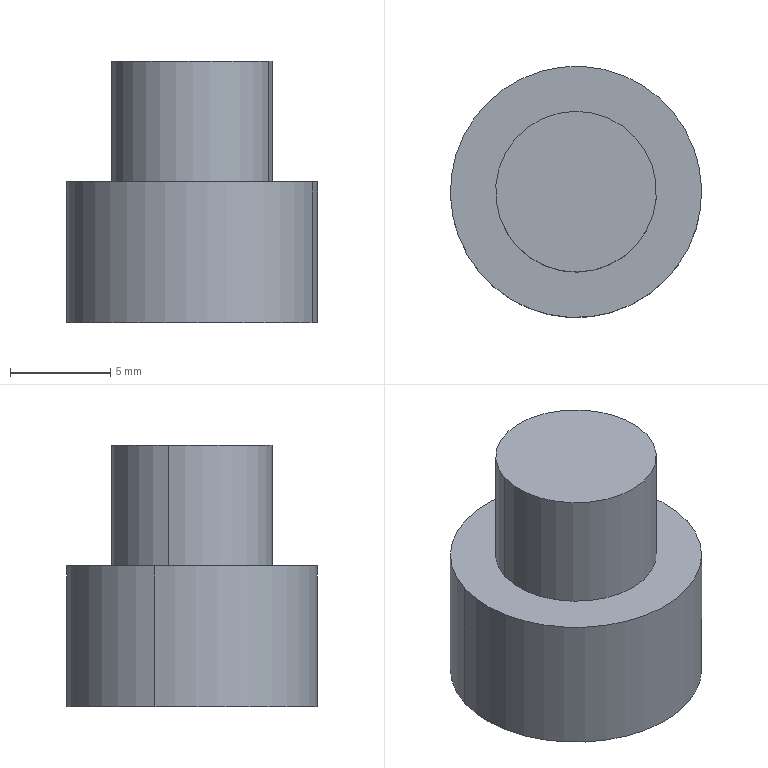Component | SolidWorks | PER_N-1 | 1 solid | 7 faces | box 12.5 x 12.5 x 13 mm | volume 1161 mm3 | cylinder 4 | plane 3 | commonest cylinder face diameters 8 x2 12.5 x2
build123d program:
from build123d import *

# Parameters (mm, degrees)
IZIM1_R                     = 6.25
Y_KSEKLIK_EKSTR_ZYON1_DEPTH = 7
IZIM2_R                     = 4
Y_KSEKLIK_EKSTR_ZYON2_DEPTH = 6


with BuildPart() as part:
    # izim1 → Y_kseklik-Ekstr_zyon1 (new body)
    with BuildSketch(Plane.XY):
        Circle(IZIM1_R)
    extrude(amount=Y_KSEKLIK_EKSTR_ZYON1_DEPTH)

    # izim2 → Y_kseklik-Ekstr_zyon2 (add)
    with BuildSketch(Plane.XY.offset(7)):
        Circle(IZIM2_R)
    extrude(amount=Y_KSEKLIK_EKSTR_ZYON2_DEPTH)


solid = part.part

# Placed as in the assembly
solid = solid.moved(Location((-146.473, 169.805, 173.974), (0, 0, 0)))
STEP:
#1=COLOUR_RGB('',0.7922,0.8196,0.9333);
#2=FILL_AREA_STYLE_COLOUR('',#1);
#3=FILL_AREA_STYLE('',(#2));
#4=SURFACE_STYLE_FILL_AREA(#3);
#5=SURFACE_SIDE_STYLE('',(#4));
#6=SURFACE_STYLE_USAGE(.BOTH.,#5);
#7=PRESENTATION_STYLE_ASSIGNMENT((#6));
#8=CARTESIAN_POINT('',(-5.917,6.732,7.361));
#9=VERTEX_POINT('',#8);
#10=CARTESIAN_POINT('',(-5.616,6.639,7.361));
#11=VERTEX_POINT('',#10);
#12=CARTESIAN_POINT('',(-5.767,6.685,7.361));
#13=DIRECTION('',(-0.,0.,1.));
#14=DIRECTION('',(-0.9556,0.2947,0.));
#15=AXIS2_PLACEMENT_3D('',#12,#13,#14);
#16=CIRCLE('',#15,0.1575);
#17=EDGE_CURVE('',#9,#11,#16,.T.);
#18=ORIENTED_EDGE('',*,*,#17,.F.);
#19=CARTESIAN_POINT('',(-5.917,6.732,7.125));
#20=VERTEX_POINT('',#19);
#21=CARTESIAN_POINT('',(-5.917,6.732,7.361));
#22=DIRECTION('',(0.,-0.,-1.));
#23=VECTOR('',#22,39.37);
#24=LINE('',#21,#23);
#25=EDGE_CURVE('',#9,#20,#24,.T.);
#26=ORIENTED_EDGE('',*,*,#25,.T.);
#27=CARTESIAN_POINT('',(-5.616,6.639,7.125));
#28=VERTEX_POINT('',#27);
#29=CARTESIAN_POINT('',(-5.767,6.685,7.125));
#30=DIRECTION('',(-0.,0.,1.));
#31=DIRECTION('',(-0.9556,0.2947,0.));
#32=AXIS2_PLACEMENT_3D('',#29,#30,#31);
#33=CIRCLE('',#32,0.1575);
#34=EDGE_CURVE('',#20,#28,#33,.T.);
#35=ORIENTED_EDGE('',*,*,#34,.T.);
#36=CARTESIAN_POINT('',(-5.616,6.639,7.361));
#37=DIRECTION('',(0.,-0.,-1.));
#38=VECTOR('',#37,39.37);
#39=LINE('',#36,#38);
#40=EDGE_CURVE('',#11,#28,#39,.T.);
#41=ORIENTED_EDGE('',*,*,#40,.F.);
#42=EDGE_LOOP('',(#18,#26,#35,#41));
#43=FACE_OUTER_BOUND('',#42,.T.);
#44=CARTESIAN_POINT('',(-5.767,6.685,7.361));
#45=DIRECTION('',(0.,-0.,-1.));
#46=DIRECTION('',(0.9556,-0.2947,0.));
#47=AXIS2_PLACEMENT_3D('',#44,#45,#46);
#48=CYLINDRICAL_SURFACE('',#47,0.1575);
#49=ADVANCED_FACE('',(#43),#48,.T.);
#50=CARTESIAN_POINT('',(-6.002,6.758,7.125));
#51=VERTEX_POINT('',#50);
#52=CARTESIAN_POINT('',(-5.532,6.613,7.125));
#53=VERTEX_POINT('',#52);
#54=CARTESIAN_POINT('',(-5.767,6.685,7.125));
#55=DIRECTION('',(-0.,0.,1.));
#56=DIRECTION('',(-0.9556,0.2947,0.));
#57=AXIS2_PLACEMENT_3D('',#54,#55,#56);
#58=CIRCLE('',#57,0.2461);
#59=EDGE_CURVE('',#51,#53,#58,.T.);
#60=ORIENTED_EDGE('',*,*,#59,.F.);
#61=CARTESIAN_POINT('',(-6.002,6.758,6.849));
#62=VERTEX_POINT('',#61);
#63=CARTESIAN_POINT('',(-6.002,6.758,7.125));
#64=DIRECTION('',(0.,-0.,-1.));
#65=VECTOR('',#64,39.37);
#66=LINE('',#63,#65);
#67=EDGE_CURVE('',#51,#62,#66,.T.);
#68=ORIENTED_EDGE('',*,*,#67,.T.);
#69=CARTESIAN_POINT('',(-5.532,6.613,6.849));
#70=VERTEX_POINT('',#69);
#71=CARTESIAN_POINT('',(-5.767,6.685,6.849));
#72=DIRECTION('',(-0.,0.,1.));
#73=DIRECTION('',(-0.9556,0.2947,0.));
#74=AXIS2_PLACEMENT_3D('',#71,#72,#73);
#75=CIRCLE('',#74,0.2461);
#76=EDGE_CURVE('',#62,#70,#75,.T.);
#77=ORIENTED_EDGE('',*,*,#76,.T.);
#78=CARTESIAN_POINT('',(-5.532,6.613,7.125));
#79=DIRECTION('',(0.,-0.,-1.));
#80=VECTOR('',#79,39.37);
#81=LINE('',#78,#80);
#82=EDGE_CURVE('',#53,#70,#81,.T.);
#83=ORIENTED_EDGE('',*,*,#82,.F.);
#84=EDGE_LOOP('',(#60,#68,#77,#83));
#85=FACE_OUTER_BOUND('',#84,.T.);
#86=CARTESIAN_POINT('',(-5.767,6.685,7.125));
#87=DIRECTION('',(0.,-0.,-1.));
#88=DIRECTION('',(0.9556,-0.2947,0.));
#89=AXIS2_PLACEMENT_3D('',#86,#87,#88);
#90=CYLINDRICAL_SURFACE('',#89,0.2461);
#91=ADVANCED_FACE('',(#85),#90,.T.);
#92=ORIENTED_EDGE('',*,*,#67,.F.);
#93=CARTESIAN_POINT('',(-5.767,6.685,7.125));
#94=DIRECTION('',(-0.,0.,1.));
#95=DIRECTION('',(-0.9556,0.2947,0.));
#96=AXIS2_PLACEMENT_3D('',#93,#94,#95);
#97=CIRCLE('',#96,0.2461);
#98=EDGE_CURVE('',#53,#51,#97,.T.);
#99=ORIENTED_EDGE('',*,*,#98,.F.);
#100=ORIENTED_EDGE('',*,*,#82,.T.);
#101=CARTESIAN_POINT('',(-5.767,6.685,6.849));
#102=DIRECTION('',(-0.,0.,1.));
#103=DIRECTION('',(-0.9556,0.2947,0.));
#104=AXIS2_PLACEMENT_3D('',#101,#102,#103);
#105=CIRCLE('',#104,0.2461);
#106=EDGE_CURVE('',#70,#62,#105,.T.);
#107=ORIENTED_EDGE('',*,*,#106,.T.);
#108=EDGE_LOOP('',(#92,#99,#100,#107));
#109=FACE_OUTER_BOUND('',#108,.T.);
#110=CARTESIAN_POINT('',(-5.767,6.685,7.125));
#111=DIRECTION('',(0.,-0.,-1.));
#112=DIRECTION('',(0.9556,-0.2947,0.));
#113=AXIS2_PLACEMENT_3D('',#110,#111,#112);
#114=CYLINDRICAL_SURFACE('',#113,0.2461);
#115=ADVANCED_FACE('',(#109),#114,.T.);
#116=CARTESIAN_POINT('',(-5.767,6.685,7.125));
#117=DIRECTION('',(-0.,0.,1.));
#118=DIRECTION('',(-0.9556,0.2947,0.));
#119=AXIS2_PLACEMENT_3D('',#116,#117,#118);
#120=CIRCLE('',#119,0.1575);
#121=EDGE_CURVE('',#28,#20,#120,.T.);
#122=ORIENTED_EDGE('',*,*,#121,.F.);
#123=ORIENTED_EDGE('',*,*,#34,.F.);
#124=EDGE_LOOP('',(#122,#123));
#125=FACE_BOUND('',#124,.T.);
#126=ORIENTED_EDGE('',*,*,#98,.T.);
#127=ORIENTED_EDGE('',*,*,#59,.T.);
#128=EDGE_LOOP('',(#126,#127));
#129=FACE_OUTER_BOUND('',#128,.T.);
#130=CARTESIAN_POINT('',(-5.767,6.685,7.125));
#131=DIRECTION('',(-0.,0.,1.));
#132=DIRECTION('',(-0.9556,0.2947,-0.));
#133=AXIS2_PLACEMENT_3D('',#130,#131,#132);
#134=PLANE('',#133);
#135=ADVANCED_FACE('',(#125,#129),#134,.T.);
#136=ORIENTED_EDGE('',*,*,#106,.F.);
#137=ORIENTED_EDGE('',*,*,#76,.F.);
#138=EDGE_LOOP('',(#136,#137));
#139=FACE_OUTER_BOUND('',#138,.T.);
#140=CARTESIAN_POINT('',(-5.767,6.685,6.849));
#141=DIRECTION('',(-0.,0.,1.));
#142=DIRECTION('',(-0.9556,0.2947,-0.));
#143=AXIS2_PLACEMENT_3D('',#140,#141,#142);
#144=PLANE('',#143);
#145=ADVANCED_FACE('',(#139),#144,.F.);
#146=ORIENTED_EDGE('',*,*,#25,.F.);
#147=CARTESIAN_POINT('',(-5.767,6.685,7.361));
#148=DIRECTION('',(-0.,0.,1.));
#149=DIRECTION('',(-0.9556,0.2947,0.));
#150=AXIS2_PLACEMENT_3D('',#147,#148,#149);
#151=CIRCLE('',#150,0.1575);
#152=EDGE_CURVE('',#11,#9,#151,.T.);
#153=ORIENTED_EDGE('',*,*,#152,.F.);
#154=ORIENTED_EDGE('',*,*,#40,.T.);
#155=ORIENTED_EDGE('',*,*,#121,.T.);
#156=EDGE_LOOP('',(#146,#153,#154,#155));
#157=FACE_OUTER_BOUND('',#156,.T.);
#158=CARTESIAN_POINT('',(-5.767,6.685,7.361));
#159=DIRECTION('',(0.,-0.,-1.));
#160=DIRECTION('',(0.9556,-0.2947,0.));
#161=AXIS2_PLACEMENT_3D('',#158,#159,#160);
#162=CYLINDRICAL_SURFACE('',#161,0.1575);
#163=ADVANCED_FACE('',(#157),#162,.T.);
#164=ORIENTED_EDGE('',*,*,#152,.T.);
#165=ORIENTED_EDGE('',*,*,#17,.T.);
#166=EDGE_LOOP('',(#164,#165));
#167=FACE_OUTER_BOUND('',#166,.T.);
#168=CARTESIAN_POINT('',(-5.767,6.685,7.361));
#169=DIRECTION('',(-0.,0.,1.));
#170=DIRECTION('',(-0.9556,0.2947,-0.));
#171=AXIS2_PLACEMENT_3D('',#168,#169,#170);
#172=PLANE('',#171);
#173=ADVANCED_FACE('',(#167),#172,.T.);
#174=CLOSED_SHELL('',(#49,#91,#115,#135,#145,#163,#173));
#175=MANIFOLD_SOLID_BREP('',#174);
#176=STYLED_ITEM('',(#7),#175);
#177=PRESENTATION_LAYER_ASSIGNMENT('','',(#176));
#178=CARTESIAN_POINT('',(0.,0.,0.));
#179=DIRECTION('',(0.,0.,1.));
#180=DIRECTION('',(1.,0.,0.));
#181=AXIS2_PLACEMENT_3D('',#178,#179,#180);
#182=(LENGTH_UNIT()NAMED_UNIT(*)SI_UNIT($,.METRE.));
#183=LENGTH_MEASURE_WITH_UNIT(LENGTH_MEASURE(0.0254),#182);
#184=DIMENSIONAL_EXPONENTS(1.,0.,0.,0.,0.,0.,0.);
#185=(CONVERSION_BASED_UNIT('',#183)LENGTH_UNIT()NAMED_UNIT(#184));
#186=UNCERTAINTY_MEASURE_WITH_UNIT(LENGTH_MEASURE(0.00001),#185,'','');
#187=(NAMED_UNIT(*)PLANE_ANGLE_UNIT()SI_UNIT($,.RADIAN.));
#188=(NAMED_UNIT(*)SI_UNIT($,.STERADIAN.)SOLID_ANGLE_UNIT());
#189=(GEOMETRIC_REPRESENTATION_CONTEXT(3)GLOBAL_UNCERTAINTY_ASSIGNED_CONTEXT((#186))GLOBAL_UNIT_ASSIGNED_CONTEXT((#185,#187,#188))REPRESENTATION_CONTEXT('',''));
#190=ADVANCED_BREP_SHAPE_REPRESENTATION('',(#175,#181),#189);
#191=(LENGTH_UNIT()NAMED_UNIT(*)SI_UNIT($,.METRE.));
#192=LENGTH_MEASURE_WITH_UNIT(LENGTH_MEASURE(0.0254),#191);
#193=DIMENSIONAL_EXPONENTS(1.,0.,0.,0.,0.,0.,0.);
#194=(CONVERSION_BASED_UNIT('',#192)LENGTH_UNIT()NAMED_UNIT(#193));
#195=UNCERTAINTY_MEASURE_WITH_UNIT(LENGTH_MEASURE(0.00001),#194,'','');
#196=(NAMED_UNIT(*)PLANE_ANGLE_UNIT()SI_UNIT($,.RADIAN.));
#197=(NAMED_UNIT(*)SI_UNIT($,.STERADIAN.)SOLID_ANGLE_UNIT());
#198=(GEOMETRIC_REPRESENTATION_CONTEXT(3)GLOBAL_UNCERTAINTY_ASSIGNED_CONTEXT((#195))GLOBAL_UNIT_ASSIGNED_CONTEXT((#194,#196,#197))REPRESENTATION_CONTEXT('',''));
#199=MECHANICAL_DESIGN_GEOMETRIC_PRESENTATION_REPRESENTATION('',(#176),#198);